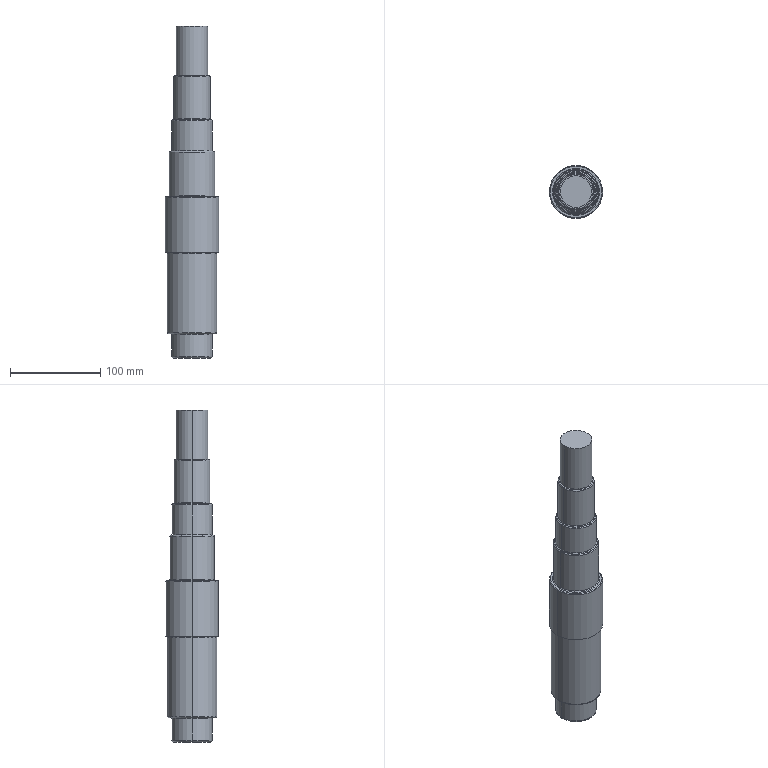Component | SolidWorks | AxisOne-1 | 1 solid | 44 faces | box 59 x 59 x 368 mm | volume 694478 mm3 | torus 22 | cylinder 14 | plane 8 | commonest cylinder face diameters 45 x4 35 x2 40 x2 50 x2 59 x2 55 x2
build123d program:
from build123d import *


with BuildPart() as part:
    # Sketch1 → Revolve1 (revolve)
    with BuildSketch(Plane(origin=(0, 0, 0), x_dir=(0, 0, -1), z_dir=(1, 0, 0)), mode=Mode.PRIVATE) as revolve1_sk:
        with BuildLine():
            Line((0, 0), (0, 17.5))
            Line((0, 17.5), (55, 17.5))
            Line((55, 17.5), (55, 19))
            ThreePointArc((55, 19), (55.293, 19.707), (56, 20))
            Line((56, 20), (103, 20))
            ThreePointArc((103, 20), (103.707, 20.293), (104, 21))
            Line((104, 21), (104, 21.5))
            ThreePointArc((104, 21.5), (104.293, 22.207), (105, 22.5))
            Line((105, 22.5), (138, 22.5))
            ThreePointArc((138, 22.5), (138.707, 22.793), (139, 23.5))
            Line((139, 23.5), (139, 24))
            ThreePointArc((139, 24), (139.293, 24.707), (140, 25))
            Line((140, 25), (188, 25))
            ThreePointArc((188, 25), (188.707, 25.293), (189, 26))
            Line((189, 26), (189, 28.5))
            ThreePointArc((189, 28.5), (189.293, 29.207), (190, 29.5))
            Line((190, 29.5), (251, 29.5))
            Line((251, 29.5), (251, 28.5))
            ThreePointArc((251, 28.5), (251.293, 27.793), (252, 27.5))
            Line((252, 27.5), (340, 27.5))
            ThreePointArc((340, 27.5), (340.707, 27.207), (341, 26.5))
            Line((341, 26.5), (341, 23.5))
            ThreePointArc((341, 23.5), (341.293, 22.793), (342, 22.5))
            Line((342, 22.5), (366, 22.5))
            ThreePointArc((366, 22.5), (367.414, 21.914), (368, 20.5))
            Line((368, 20.5), (368, 0))
            Line((368, 0), (0, 0))
        make_face()
    revolve(revolve1_sk.sketch.rotate(Axis((0, 0, -368), (0, 0, 1)), 90), axis=Axis((0, 0, -368), (0, 0, 1)))


solid = part.part

# Placed as in the assembly
solid = solid.moved(Location((35.733, 15.31, 121.5), (0, 0, 0)))